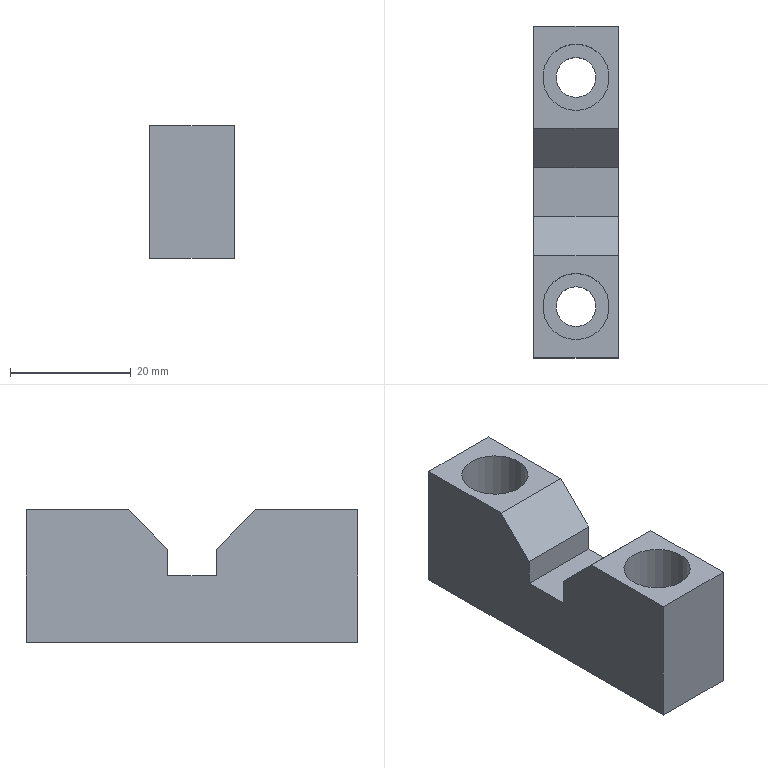Component | NX | FIXED_V_BLOCK | 1 solid | 18 faces | volume 11922 mm3 | plane 14 | cylinder 4 | commonest cylinder face diameters 6.6 x2 11 x2